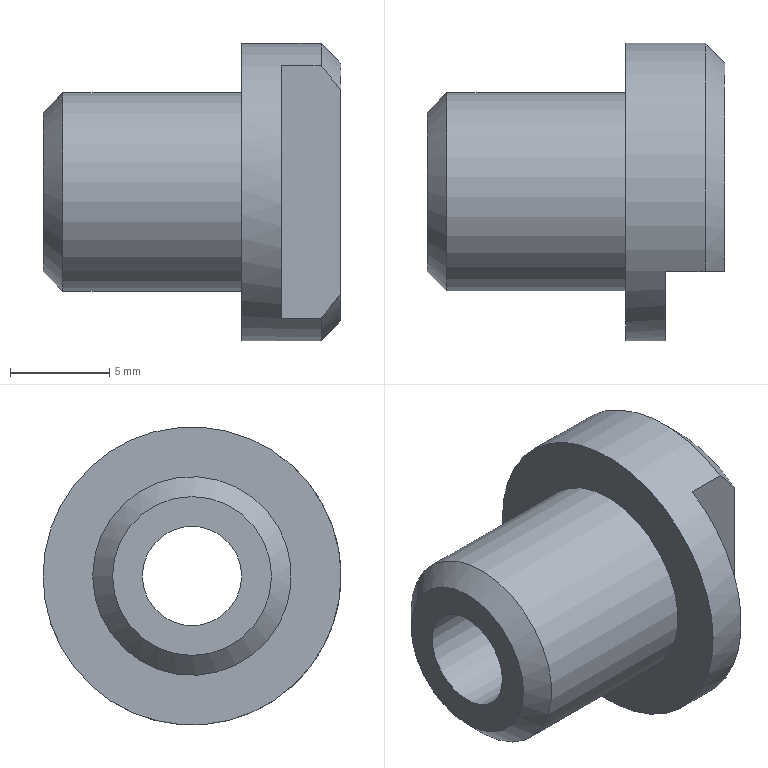Component | NX | DRILL_BUSHING | 1 solid | 10 faces | box 15 x 15 x 15 mm | volume 1250 mm3 | plane 5 | cylinder 3 | cone 2 | commonest cylinder face diameters 10 x1 15 x1 5 x1
STEP:
#1=CARTESIAN_POINT('',(0.,0.,0.));
#2=DIRECTION('',(0.,0.,1.));
#3=DIRECTION('',(1.,0.,0.));
#4=AXIS2_PLACEMENT_3D('',#1,#2,#3);
#5=CARTESIAN_POINT('',(50.511,134.396,30.));
#6=VERTEX_POINT('',#5);
#7=CARTESIAN_POINT('',(50.511,129.396,30.));
#8=DIRECTION('',(1.,0.,0.));
#9=DIRECTION('',(0.,1.,0.));
#10=AXIS2_PLACEMENT_3D('',#7,#8,#9);
#11=CIRCLE('',#10,5.);
#12=CARTESIAN_POINT('',(59.511,129.396,30.));
#13=DIRECTION('',(-1.,0.,0.));
#14=DIRECTION('',(0.,-1.,0.));
#15=AXIS2_PLACEMENT_3D('',#12,#13,#14);
#16=CYLINDRICAL_SURFACE('',#15,5.);
#17=CARTESIAN_POINT('',(9.425,9.));
#18=DIRECTION('',(-1.,0.));
#19=VECTOR('',#18,1.);
#20=LINE('',#17,#19);
#21=(GEOMETRIC_REPRESENTATION_CONTEXT(2)PARAMETRIC_REPRESENTATION_CONTEXT()REPRESENTATION_CONTEXT('',''));
#22=DEFINITIONAL_REPRESENTATION('',(#20),#21);
#23=PCURVE('',#16,#22);
#24=CARTESIAN_POINT('',(50.511,129.396,30.));
#25=DIRECTION('',(1.,0.,0.));
#26=DIRECTION('',(0.,1.,0.));
#27=AXIS2_PLACEMENT_3D('',#24,#25,#26);
#28=CONICAL_SURFACE('',#27,5.,0.7854);
#29=CARTESIAN_POINT('',(0.,0.));
#30=DIRECTION('',(1.,0.));
#31=VECTOR('',#30,1.);
#32=LINE('',#29,#31);
#33=(GEOMETRIC_REPRESENTATION_CONTEXT(2)PARAMETRIC_REPRESENTATION_CONTEXT()REPRESENTATION_CONTEXT('',''));
#34=DEFINITIONAL_REPRESENTATION('',(#32),#33);
#35=PCURVE('',#28,#34);
#36=SURFACE_CURVE('',#11,(#23,#35),.PCURVE_S1.);
#37=EDGE_CURVE('',#6,#6,#36,.T.);
#38=ORIENTED_EDGE('',*,*,#37,.T.);
#39=CARTESIAN_POINT('',(59.511,134.396,30.));
#40=VERTEX_POINT('',#39);
#41=CARTESIAN_POINT('',(59.511,134.396,30.));
#42=CARTESIAN_POINT('',(50.511,134.396,30.));
#43=B_SPLINE_CURVE_WITH_KNOTS('',1,(#41,#42),.UNSPECIFIED.,.F.,.F.,(2,2),(0.,9.),.PIECEWISE_BEZIER_KNOTS.);
#44=CARTESIAN_POINT('',(3.142,0.));
#45=DIRECTION('',(0.,1.));
#46=VECTOR('',#45,1.);
#47=LINE('',#44,#46);
#48=(GEOMETRIC_REPRESENTATION_CONTEXT(2)PARAMETRIC_REPRESENTATION_CONTEXT()REPRESENTATION_CONTEXT('',''));
#49=DEFINITIONAL_REPRESENTATION('',(#47),#48);
#50=PCURVE('',#16,#49);
#51=CARTESIAN_POINT('',(9.425,0.));
#52=DIRECTION('',(0.,1.));
#53=VECTOR('',#52,1.);
#54=LINE('',#51,#53);
#55=(GEOMETRIC_REPRESENTATION_CONTEXT(2)PARAMETRIC_REPRESENTATION_CONTEXT()REPRESENTATION_CONTEXT('',''));
#56=DEFINITIONAL_REPRESENTATION('',(#54),#55);
#57=PCURVE('',#16,#56);
#58=SEAM_CURVE('',#43,(#50,#57),.PCURVE_S1.);
#59=EDGE_CURVE('',#40,#6,#58,.T.);
#60=ORIENTED_EDGE('',*,*,#59,.F.);
#61=CARTESIAN_POINT('',(59.511,129.396,30.));
#62=DIRECTION('',(1.,0.,0.));
#63=DIRECTION('',(0.,1.,0.));
#64=AXIS2_PLACEMENT_3D('',#61,#62,#63);
#65=CIRCLE('',#64,5.);
#66=CARTESIAN_POINT('',(9.425,0.));
#67=DIRECTION('',(-1.,0.));
#68=VECTOR('',#67,1.);
#69=LINE('',#66,#68);
#70=(GEOMETRIC_REPRESENTATION_CONTEXT(2)PARAMETRIC_REPRESENTATION_CONTEXT()REPRESENTATION_CONTEXT('',''));
#71=DEFINITIONAL_REPRESENTATION('',(#69),#70);
#72=PCURVE('',#16,#71);
#73=CARTESIAN_POINT('',(59.511,129.396,30.));
#74=DIRECTION('',(1.,0.,0.));
#75=DIRECTION('',(0.,1.,0.));
#76=AXIS2_PLACEMENT_3D('',#73,#74,#75);
#77=PLANE('',#76);
#78=CARTESIAN_POINT('',(0.,0.));
#79=DIRECTION('',(1.,0.));
#80=AXIS2_PLACEMENT_2D('',#78,#79);
#81=CIRCLE('',#80,5.);
#82=(GEOMETRIC_REPRESENTATION_CONTEXT(2)PARAMETRIC_REPRESENTATION_CONTEXT()REPRESENTATION_CONTEXT('',''));
#83=DEFINITIONAL_REPRESENTATION('',(#81),#82);
#84=PCURVE('',#77,#83);
#85=SURFACE_CURVE('',#65,(#72,#84),.PCURVE_S1.);
#86=EDGE_CURVE('',#40,#40,#85,.T.);
#87=ORIENTED_EDGE('',*,*,#86,.F.);
#88=ORIENTED_EDGE('',*,*,#59,.T.);
#89=EDGE_LOOP('',(#38,#60,#87,#88));
#90=FACE_BOUND('',#89,.T.);
#91=ADVANCED_FACE('',(#90),#16,.T.);
#92=CARTESIAN_POINT('',(49.511,133.396,30.));
#93=VERTEX_POINT('',#92);
#94=CARTESIAN_POINT('',(49.511,129.396,30.));
#95=DIRECTION('',(-1.,0.,0.));
#96=DIRECTION('',(0.,1.,0.));
#97=AXIS2_PLACEMENT_3D('',#94,#95,#96);
#98=CIRCLE('',#97,4.);
#99=CARTESIAN_POINT('',(49.511,129.396,30.));
#100=DIRECTION('',(1.,0.,0.));
#101=DIRECTION('',(0.,1.,0.));
#102=AXIS2_PLACEMENT_3D('',#99,#100,#101);
#103=PLANE('',#102);
#104=CARTESIAN_POINT('',(4.,0.));
#105=CARTESIAN_POINT('',(4.,-6.928));
#106=CARTESIAN_POINT('',(-2.,-3.464));
#107=CARTESIAN_POINT('',(-8.,-0.));
#108=CARTESIAN_POINT('',(-2.,3.464));
#109=CARTESIAN_POINT('',(4.,6.928));
#110=CARTESIAN_POINT('',(4.,0.));
#111=(BOUNDED_CURVE()B_SPLINE_CURVE(2,(#104,#105,#106,#107,#108,#109,#110),.UNSPECIFIED.,.T.,.F.)B_SPLINE_CURVE_WITH_KNOTS((1,2,2,2,2,1),(-2.094,0.,2.094,4.189,6.283,8.378),.UNSPECIFIED.)CURVE()GEOMETRIC_REPRESENTATION_ITEM()RATIONAL_B_SPLINE_CURVE((1.,0.5,1.,0.5,1.,0.5,1.))REPRESENTATION_ITEM(''));
#112=(GEOMETRIC_REPRESENTATION_CONTEXT(2)PARAMETRIC_REPRESENTATION_CONTEXT()REPRESENTATION_CONTEXT('',''));
#113=DEFINITIONAL_REPRESENTATION('',(#111),#112);
#114=PCURVE('',#103,#113);
#115=CARTESIAN_POINT('',(6.283,-1.));
#116=DIRECTION('',(-1.,0.));
#117=VECTOR('',#116,1.);
#118=LINE('',#115,#117);
#119=(GEOMETRIC_REPRESENTATION_CONTEXT(2)PARAMETRIC_REPRESENTATION_CONTEXT()REPRESENTATION_CONTEXT('',''));
#120=DEFINITIONAL_REPRESENTATION('',(#118),#119);
#121=PCURVE('',#28,#120);
#122=SURFACE_CURVE('',#98,(#114,#121),.PCURVE_S1.);
#123=EDGE_CURVE('',#93,#93,#122,.T.);
#124=ORIENTED_EDGE('',*,*,#123,.T.);
#125=EDGE_LOOP('',(#124));
#126=FACE_BOUND('',#125,.T.);
#127=CARTESIAN_POINT('',(49.511,131.896,30.));
#128=VERTEX_POINT('',#127);
#129=CARTESIAN_POINT('',(49.511,129.396,30.));
#130=DIRECTION('',(1.,0.,0.));
#131=DIRECTION('',(0.,1.,0.));
#132=AXIS2_PLACEMENT_3D('',#129,#130,#131);
#133=CIRCLE('',#132,2.5);
#134=CARTESIAN_POINT('',(0.,0.));
#135=DIRECTION('',(1.,0.));
#136=AXIS2_PLACEMENT_2D('',#134,#135);
#137=CIRCLE('',#136,2.5);
#138=(GEOMETRIC_REPRESENTATION_CONTEXT(2)PARAMETRIC_REPRESENTATION_CONTEXT()REPRESENTATION_CONTEXT('',''));
#139=DEFINITIONAL_REPRESENTATION('',(#137),#138);
#140=PCURVE('',#103,#139);
#141=CARTESIAN_POINT('',(46.211,129.396,30.));
#142=DIRECTION('',(1.,0.,0.));
#143=DIRECTION('',(0.,1.,0.));
#144=AXIS2_PLACEMENT_3D('',#141,#142,#143);
#145=CYLINDRICAL_SURFACE('',#144,2.5);
#146=CARTESIAN_POINT('',(0.,3.3));
#147=DIRECTION('',(1.,0.));
#148=VECTOR('',#147,1.);
#149=LINE('',#146,#148);
#150=(GEOMETRIC_REPRESENTATION_CONTEXT(2)PARAMETRIC_REPRESENTATION_CONTEXT()REPRESENTATION_CONTEXT('',''));
#151=DEFINITIONAL_REPRESENTATION('',(#149),#150);
#152=PCURVE('',#145,#151);
#153=SURFACE_CURVE('',#133,(#140,#152),.PCURVE_S1.);
#154=EDGE_CURVE('',#128,#128,#153,.T.);
#155=ORIENTED_EDGE('',*,*,#154,.T.);
#156=EDGE_LOOP('',(#155));
#157=FACE_BOUND('',#156,.T.);
#158=ADVANCED_FACE('',(#126,#157),#103,.F.);
#159=CARTESIAN_POINT('',(63.511,125.396,36.344));
#160=VERTEX_POINT('',#159);
#161=CARTESIAN_POINT('',(63.511,125.396,23.656));
#162=VERTEX_POINT('',#161);
#163=CARTESIAN_POINT('',(63.511,129.396,30.));
#164=DIRECTION('',(-1.,0.,0.));
#165=DIRECTION('',(0.,1.,0.));
#166=AXIS2_PLACEMENT_3D('',#163,#164,#165);
#167=CIRCLE('',#166,7.5);
#168=CARTESIAN_POINT('',(64.511,129.396,30.));
#169=DIRECTION('',(-1.,0.,0.));
#170=DIRECTION('',(0.,-1.,0.));
#171=AXIS2_PLACEMENT_3D('',#168,#169,#170);
#172=CYLINDRICAL_SURFACE('',#171,7.5);
#173=CARTESIAN_POINT('',(-3.142,1.));
#174=DIRECTION('',(1.,0.));
#175=VECTOR('',#174,1.);
#176=LINE('',#173,#175);
#177=(GEOMETRIC_REPRESENTATION_CONTEXT(2)PARAMETRIC_REPRESENTATION_CONTEXT()REPRESENTATION_CONTEXT('',''));
#178=DEFINITIONAL_REPRESENTATION('',(#176),#177);
#179=PCURVE('',#172,#178);
#180=CARTESIAN_POINT('',(64.511,129.396,30.));
#181=DIRECTION('',(-1.,0.,0.));
#182=DIRECTION('',(0.,-1.,0.));
#183=AXIS2_PLACEMENT_3D('',#180,#181,#182);
#184=CONICAL_SURFACE('',#183,6.5,0.7854);
#185=CARTESIAN_POINT('',(-3.142,1.));
#186=DIRECTION('',(1.,0.));
#187=VECTOR('',#186,1.);
#188=LINE('',#185,#187);
#189=(GEOMETRIC_REPRESENTATION_CONTEXT(2)PARAMETRIC_REPRESENTATION_CONTEXT()REPRESENTATION_CONTEXT('',''));
#190=DEFINITIONAL_REPRESENTATION('',(#188),#189);
#191=PCURVE('',#184,#190);
#192=SURFACE_CURVE('',#167,(#179,#191),.PCURVE_S1.);
#193=EDGE_CURVE('',#160,#162,#192,.T.);
#194=ORIENTED_EDGE('',*,*,#193,.T.);
#195=CARTESIAN_POINT('',(61.511,125.396,23.656));
#196=VERTEX_POINT('',#195);
#197=CARTESIAN_POINT('',(64.511,125.396,23.656));
#198=DIRECTION('',(-1.,0.,0.));
#199=VECTOR('',#198,1.);
#200=LINE('',#197,#199);
#201=CARTESIAN_POINT('',(5.275,0.));
#202=DIRECTION('',(0.,1.));
#203=VECTOR('',#202,1.);
#204=LINE('',#201,#203);
#205=(GEOMETRIC_REPRESENTATION_CONTEXT(2)PARAMETRIC_REPRESENTATION_CONTEXT()REPRESENTATION_CONTEXT('',''));
#206=DEFINITIONAL_REPRESENTATION('',(#204),#205);
#207=PCURVE('',#172,#206);
#208=CARTESIAN_POINT('',(61.511,125.396,22.2));
#209=DIRECTION('',(0.,1.,0.));
#210=DIRECTION('',(0.,-0.,1.));
#211=AXIS2_PLACEMENT_3D('',#208,#209,#210);
#212=PLANE('',#211);
#213=CARTESIAN_POINT('',(1.456,3.));
#214=DIRECTION('',(0.,-1.));
#215=VECTOR('',#214,1.);
#216=LINE('',#213,#215);
#217=(GEOMETRIC_REPRESENTATION_CONTEXT(2)PARAMETRIC_REPRESENTATION_CONTEXT()REPRESENTATION_CONTEXT('',''));
#218=DEFINITIONAL_REPRESENTATION('',(#216),#217);
#219=PCURVE('',#212,#218);
#220=SURFACE_CURVE('',#200,(#207,#219),.PCURVE_S1.);
#221=EDGE_CURVE('',#162,#196,#220,.T.);
#222=ORIENTED_EDGE('',*,*,#221,.T.);
#223=CARTESIAN_POINT('',(61.511,125.396,36.344));
#224=VERTEX_POINT('',#223);
#225=CARTESIAN_POINT('',(61.511,129.396,30.));
#226=DIRECTION('',(1.,0.,0.));
#227=DIRECTION('',(0.,1.,0.));
#228=AXIS2_PLACEMENT_3D('',#225,#226,#227);
#229=CIRCLE('',#228,7.5);
#230=CARTESIAN_POINT('',(9.425,3.));
#231=DIRECTION('',(-1.,0.));
#232=VECTOR('',#231,1.);
#233=LINE('',#230,#232);
#234=(GEOMETRIC_REPRESENTATION_CONTEXT(2)PARAMETRIC_REPRESENTATION_CONTEXT()REPRESENTATION_CONTEXT('',''));
#235=DEFINITIONAL_REPRESENTATION('',(#233),#234);
#236=PCURVE('',#172,#235);
#237=CARTESIAN_POINT('',(61.511,129.396,30.));
#238=DIRECTION('',(1.,0.,0.));
#239=DIRECTION('',(0.,1.,0.));
#240=AXIS2_PLACEMENT_3D('',#237,#238,#239);
#241=PLANE('',#240);
#242=CARTESIAN_POINT('',(0.,0.));
#243=DIRECTION('',(1.,0.));
#244=AXIS2_PLACEMENT_2D('',#242,#243);
#245=CIRCLE('',#244,7.5);
#246=(GEOMETRIC_REPRESENTATION_CONTEXT(2)PARAMETRIC_REPRESENTATION_CONTEXT()REPRESENTATION_CONTEXT('',''));
#247=DEFINITIONAL_REPRESENTATION('',(#245),#246);
#248=PCURVE('',#241,#247);
#249=SURFACE_CURVE('',#229,(#236,#248),.PCURVE_S1.);
#250=EDGE_CURVE('',#224,#196,#249,.T.);
#251=ORIENTED_EDGE('',*,*,#250,.F.);
#252=CARTESIAN_POINT('',(59.511,125.396,36.344));
#253=VERTEX_POINT('',#252);
#254=CARTESIAN_POINT('',(61.511,125.396,36.344));
#255=CARTESIAN_POINT('',(59.511,125.396,36.344));
#256=B_SPLINE_CURVE_WITH_KNOTS('',1,(#254,#255),.UNSPECIFIED.,.F.,.F.,(2,2),(3.,5.),.PIECEWISE_BEZIER_KNOTS.);
#257=CARTESIAN_POINT('',(7.291,0.));
#258=DIRECTION('',(0.,1.));
#259=VECTOR('',#258,1.);
#260=LINE('',#257,#259);
#261=(GEOMETRIC_REPRESENTATION_CONTEXT(2)PARAMETRIC_REPRESENTATION_CONTEXT()REPRESENTATION_CONTEXT('',''));
#262=DEFINITIONAL_REPRESENTATION('',(#260),#261);
#263=PCURVE('',#172,#262);
#264=CARTESIAN_POINT('',(1.008,0.));
#265=DIRECTION('',(0.,1.));
#266=VECTOR('',#265,1.);
#267=LINE('',#264,#266);
#268=(GEOMETRIC_REPRESENTATION_CONTEXT(2)PARAMETRIC_REPRESENTATION_CONTEXT()REPRESENTATION_CONTEXT('',''));
#269=DEFINITIONAL_REPRESENTATION('',(#267),#268);
#270=PCURVE('',#172,#269);
#271=SEAM_CURVE('',#256,(#263,#270),.PCURVE_S1.);
#272=EDGE_CURVE('',#224,#253,#271,.T.);
#273=ORIENTED_EDGE('',*,*,#272,.T.);
#274=CARTESIAN_POINT('',(59.511,136.896,30.));
#275=VERTEX_POINT('',#274);
#276=CARTESIAN_POINT('',(59.511,129.396,30.));
#277=DIRECTION('',(1.,0.,0.));
#278=DIRECTION('',(0.,1.,0.));
#279=AXIS2_PLACEMENT_3D('',#276,#277,#278);
#280=CIRCLE('',#279,7.5);
#281=CARTESIAN_POINT('',(9.425,5.));
#282=DIRECTION('',(-1.,0.));
#283=VECTOR('',#282,1.);
#284=LINE('',#281,#283);
#285=(GEOMETRIC_REPRESENTATION_CONTEXT(2)PARAMETRIC_REPRESENTATION_CONTEXT()REPRESENTATION_CONTEXT('',''));
#286=DEFINITIONAL_REPRESENTATION('',(#284),#285);
#287=PCURVE('',#172,#286);
#288=CARTESIAN_POINT('',(0.,0.));
#289=DIRECTION('',(1.,0.));
#290=AXIS2_PLACEMENT_2D('',#288,#289);
#291=CIRCLE('',#290,7.5);
#292=(GEOMETRIC_REPRESENTATION_CONTEXT(2)PARAMETRIC_REPRESENTATION_CONTEXT()REPRESENTATION_CONTEXT('',''));
#293=DEFINITIONAL_REPRESENTATION('',(#291),#292);
#294=PCURVE('',#77,#293);
#295=SURFACE_CURVE('',#280,(#287,#294),.PCURVE_S1.);
#296=EDGE_CURVE('',#253,#275,#295,.T.);
#297=ORIENTED_EDGE('',*,*,#296,.T.);
#298=CARTESIAN_POINT('',(59.511,129.396,30.));
#299=DIRECTION('',(1.,0.,0.));
#300=DIRECTION('',(0.,1.,0.));
#301=AXIS2_PLACEMENT_3D('',#298,#299,#300);
#302=CIRCLE('',#301,7.5);
#303=CARTESIAN_POINT('',(3.142,5.));
#304=DIRECTION('',(-1.,0.));
#305=VECTOR('',#304,1.);
#306=LINE('',#303,#305);
#307=(GEOMETRIC_REPRESENTATION_CONTEXT(2)PARAMETRIC_REPRESENTATION_CONTEXT()REPRESENTATION_CONTEXT('',''));
#308=DEFINITIONAL_REPRESENTATION('',(#306),#307);
#309=PCURVE('',#172,#308);
#310=CARTESIAN_POINT('',(0.,0.));
#311=DIRECTION('',(1.,0.));
#312=AXIS2_PLACEMENT_2D('',#310,#311);
#313=CIRCLE('',#312,7.5);
#314=(GEOMETRIC_REPRESENTATION_CONTEXT(2)PARAMETRIC_REPRESENTATION_CONTEXT()REPRESENTATION_CONTEXT('',''));
#315=DEFINITIONAL_REPRESENTATION('',(#313),#314);
#316=PCURVE('',#77,#315);
#317=SURFACE_CURVE('',#302,(#309,#316),.PCURVE_S1.);
#318=EDGE_CURVE('',#275,#253,#317,.T.);
#319=ORIENTED_EDGE('',*,*,#318,.T.);
#320=ORIENTED_EDGE('',*,*,#272,.F.);
#321=CARTESIAN_POINT('',(64.511,125.396,36.344));
#322=DIRECTION('',(1.,0.,0.));
#323=VECTOR('',#322,1.);
#324=LINE('',#321,#323);
#325=CARTESIAN_POINT('',(1.008,0.));
#326=DIRECTION('',(0.,-1.));
#327=VECTOR('',#326,1.);
#328=LINE('',#325,#327);
#329=(GEOMETRIC_REPRESENTATION_CONTEXT(2)PARAMETRIC_REPRESENTATION_CONTEXT()REPRESENTATION_CONTEXT('',''));
#330=DEFINITIONAL_REPRESENTATION('',(#328),#329);
#331=PCURVE('',#172,#330);
#332=CARTESIAN_POINT('',(14.144,3.));
#333=DIRECTION('',(0.,1.));
#334=VECTOR('',#333,1.);
#335=LINE('',#332,#334);
#336=(GEOMETRIC_REPRESENTATION_CONTEXT(2)PARAMETRIC_REPRESENTATION_CONTEXT()REPRESENTATION_CONTEXT('',''));
#337=DEFINITIONAL_REPRESENTATION('',(#335),#336);
#338=PCURVE('',#212,#337);
#339=SURFACE_CURVE('',#324,(#331,#338),.PCURVE_S1.);
#340=EDGE_CURVE('',#224,#160,#339,.T.);
#341=ORIENTED_EDGE('',*,*,#340,.T.);
#342=EDGE_LOOP('',(#194,#222,#251,#273,#297,#319,#320,#341));
#343=FACE_BOUND('',#342,.T.);
#344=ADVANCED_FACE('',(#343),#172,.T.);
#345=CARTESIAN_POINT('',(64.511,125.396,24.877));
#346=VERTEX_POINT('',#345);
#347=CARTESIAN_POINT('',(64.511,125.396,35.123));
#348=VERTEX_POINT('',#347);
#349=CARTESIAN_POINT('',(64.511,125.396,22.2));
#350=DIRECTION('',(0.,-0.,1.));
#351=VECTOR('',#350,1.);
#352=LINE('',#349,#351);
#353=CARTESIAN_POINT('',(64.511,129.396,30.));
#354=DIRECTION('',(1.,0.,0.));
#355=DIRECTION('',(0.,1.,0.));
#356=AXIS2_PLACEMENT_3D('',#353,#354,#355);
#357=PLANE('',#356);
#358=CARTESIAN_POINT('',(-4.,-7.8));
#359=DIRECTION('',(-0.,1.));
#360=VECTOR('',#359,1.);
#361=LINE('',#358,#360);
#362=(GEOMETRIC_REPRESENTATION_CONTEXT(2)PARAMETRIC_REPRESENTATION_CONTEXT()REPRESENTATION_CONTEXT('',''));
#363=DEFINITIONAL_REPRESENTATION('',(#361),#362);
#364=PCURVE('',#357,#363);
#365=CARTESIAN_POINT('',(0.,3.));
#366=DIRECTION('',(1.,0.));
#367=VECTOR('',#366,1.);
#368=LINE('',#365,#367);
#369=(GEOMETRIC_REPRESENTATION_CONTEXT(2)PARAMETRIC_REPRESENTATION_CONTEXT()REPRESENTATION_CONTEXT('',''));
#370=DEFINITIONAL_REPRESENTATION('',(#368),#369);
#371=PCURVE('',#212,#370);
#372=SURFACE_CURVE('',#352,(#364,#371),.PCURVE_S1.);
#373=EDGE_CURVE('',#346,#348,#372,.T.);
#374=ORIENTED_EDGE('',*,*,#373,.F.);
#375=CARTESIAN_POINT('',(64.511,129.396,30.));
#376=DIRECTION('',(1.,0.,0.));
#377=DIRECTION('',(0.,1.,0.));
#378=AXIS2_PLACEMENT_3D('',#375,#376,#377);
#379=CIRCLE('',#378,6.5);
#380=CARTESIAN_POINT('',(0.,0.));
#381=DIRECTION('',(1.,0.));
#382=AXIS2_PLACEMENT_2D('',#380,#381);
#383=CIRCLE('',#382,6.5);
#384=(GEOMETRIC_REPRESENTATION_CONTEXT(2)PARAMETRIC_REPRESENTATION_CONTEXT()REPRESENTATION_CONTEXT('',''));
#385=DEFINITIONAL_REPRESENTATION('',(#383),#384);
#386=PCURVE('',#357,#385);
#387=CARTESIAN_POINT('',(9.425,0.));
#388=DIRECTION('',(-1.,-0.));
#389=VECTOR('',#388,1.);
#390=LINE('',#387,#389);
#391=(GEOMETRIC_REPRESENTATION_CONTEXT(2)PARAMETRIC_REPRESENTATION_CONTEXT()REPRESENTATION_CONTEXT('',''));
#392=DEFINITIONAL_REPRESENTATION('',(#390),#391);
#393=PCURVE('',#184,#392);
#394=SURFACE_CURVE('',#379,(#386,#393),.PCURVE_S1.);
#395=EDGE_CURVE('',#346,#348,#394,.T.);
#396=ORIENTED_EDGE('',*,*,#395,.T.);
#397=EDGE_LOOP('',(#374,#396));
#398=FACE_BOUND('',#397,.T.);
#399=CARTESIAN_POINT('',(64.511,131.896,30.));
#400=VERTEX_POINT('',#399);
#401=CARTESIAN_POINT('',(64.511,129.396,30.));
#402=DIRECTION('',(1.,0.,0.));
#403=DIRECTION('',(0.,1.,0.));
#404=AXIS2_PLACEMENT_3D('',#401,#402,#403);
#405=CIRCLE('',#404,2.5);
#406=CARTESIAN_POINT('',(0.,0.));
#407=DIRECTION('',(1.,0.));
#408=AXIS2_PLACEMENT_2D('',#406,#407);
#409=CIRCLE('',#408,2.5);
#410=(GEOMETRIC_REPRESENTATION_CONTEXT(2)PARAMETRIC_REPRESENTATION_CONTEXT()REPRESENTATION_CONTEXT('',''));
#411=DEFINITIONAL_REPRESENTATION('',(#409),#410);
#412=PCURVE('',#357,#411);
#413=CARTESIAN_POINT('',(0.,18.3));
#414=DIRECTION('',(1.,0.));
#415=VECTOR('',#414,1.);
#416=LINE('',#413,#415);
#417=(GEOMETRIC_REPRESENTATION_CONTEXT(2)PARAMETRIC_REPRESENTATION_CONTEXT()REPRESENTATION_CONTEXT('',''));
#418=DEFINITIONAL_REPRESENTATION('',(#416),#417);
#419=PCURVE('',#145,#418);
#420=SURFACE_CURVE('',#405,(#412,#419),.PCURVE_S1.);
#421=EDGE_CURVE('',#400,#400,#420,.T.);
#422=ORIENTED_EDGE('',*,*,#421,.F.);
#423=EDGE_LOOP('',(#422));
#424=FACE_BOUND('',#423,.T.);
#425=ADVANCED_FACE('',(#398,#424),#357,.T.);
#426=ORIENTED_EDGE('',*,*,#86,.T.);
#427=EDGE_LOOP('',(#426));
#428=FACE_BOUND('',#427,.T.);
#429=ORIENTED_EDGE('',*,*,#318,.F.);
#430=ORIENTED_EDGE('',*,*,#296,.F.);
#431=EDGE_LOOP('',(#429,#430));
#432=FACE_BOUND('',#431,.T.);
#433=ADVANCED_FACE('',(#428,#432),#77,.F.);
#434=ORIENTED_EDGE('',*,*,#421,.F.);
#435=CARTESIAN_POINT('',(49.511,131.896,30.));
#436=CARTESIAN_POINT('',(64.511,131.896,30.));
#437=B_SPLINE_CURVE_WITH_KNOTS('',1,(#435,#436),.UNSPECIFIED.,.F.,.F.,(2,2),(3.3,18.3),.PIECEWISE_BEZIER_KNOTS.);
#438=CARTESIAN_POINT('',(0.,0.));
#439=DIRECTION('',(0.,1.));
#440=VECTOR('',#439,1.);
#441=LINE('',#438,#440);
#442=(GEOMETRIC_REPRESENTATION_CONTEXT(2)PARAMETRIC_REPRESENTATION_CONTEXT()REPRESENTATION_CONTEXT('',''));
#443=DEFINITIONAL_REPRESENTATION('',(#441),#442);
#444=PCURVE('',#145,#443);
#445=CARTESIAN_POINT('',(6.283,0.));
#446=DIRECTION('',(0.,1.));
#447=VECTOR('',#446,1.);
#448=LINE('',#445,#447);
#449=(GEOMETRIC_REPRESENTATION_CONTEXT(2)PARAMETRIC_REPRESENTATION_CONTEXT()REPRESENTATION_CONTEXT('',''));
#450=DEFINITIONAL_REPRESENTATION('',(#448),#449);
#451=PCURVE('',#145,#450);
#452=SEAM_CURVE('',#437,(#444,#451),.PCURVE_S1.);
#453=EDGE_CURVE('',#128,#400,#452,.T.);
#454=ORIENTED_EDGE('',*,*,#453,.F.);
#455=ORIENTED_EDGE('',*,*,#154,.T.);
#456=ORIENTED_EDGE('',*,*,#453,.T.);
#457=EDGE_LOOP('',(#434,#454,#455,#456));
#458=FACE_BOUND('',#457,.F.);
#459=ADVANCED_FACE('',(#458),#145,.F.);
#460=ORIENTED_EDGE('',*,*,#123,.F.);
#461=CARTESIAN_POINT('',(49.511,133.396,30.));
#462=CARTESIAN_POINT('',(50.511,134.396,30.));
#463=B_SPLINE_CURVE_WITH_KNOTS('',1,(#461,#462),.UNSPECIFIED.,.F.,.F.,(2,2),(-1.414,0.),.PIECEWISE_BEZIER_KNOTS.);
#464=CARTESIAN_POINT('',(6.283,0.));
#465=DIRECTION('',(0.,1.));
#466=VECTOR('',#465,1.);
#467=LINE('',#464,#466);
#468=(GEOMETRIC_REPRESENTATION_CONTEXT(2)PARAMETRIC_REPRESENTATION_CONTEXT()REPRESENTATION_CONTEXT('',''));
#469=DEFINITIONAL_REPRESENTATION('',(#467),#468);
#470=PCURVE('',#28,#469);
#471=CARTESIAN_POINT('',(0.,0.));
#472=DIRECTION('',(0.,1.));
#473=VECTOR('',#472,1.);
#474=LINE('',#471,#473);
#475=(GEOMETRIC_REPRESENTATION_CONTEXT(2)PARAMETRIC_REPRESENTATION_CONTEXT()REPRESENTATION_CONTEXT('',''));
#476=DEFINITIONAL_REPRESENTATION('',(#474),#475);
#477=PCURVE('',#28,#476);
#478=SEAM_CURVE('',#463,(#470,#477),.PCURVE_S1.);
#479=EDGE_CURVE('',#93,#6,#478,.T.);
#480=ORIENTED_EDGE('',*,*,#479,.T.);
#481=ORIENTED_EDGE('',*,*,#37,.F.);
#482=ORIENTED_EDGE('',*,*,#479,.F.);
#483=EDGE_LOOP('',(#460,#480,#481,#482));
#484=FACE_BOUND('',#483,.T.);
#485=ADVANCED_FACE('',(#484),#28,.T.);
#486=CARTESIAN_POINT('',(63.511,125.396,23.656));
#487=CARTESIAN_POINT('',(63.851,125.396,24.058));
#488=CARTESIAN_POINT('',(64.185,125.396,24.464));
#489=CARTESIAN_POINT('',(64.511,125.396,24.877));
#490=B_SPLINE_CURVE_WITH_KNOTS('',3,(#486,#487,#488,#489),.UNSPECIFIED.,.F.,.F.,(4,4),(0.,1.),.PIECEWISE_BEZIER_KNOTS.);
#491=CARTESIAN_POINT('',(5.275,1.));
#492=CARTESIAN_POINT('',(5.375,0.));
#493=B_SPLINE_CURVE_WITH_KNOTS('',1,(#491,#492),.UNSPECIFIED.,.F.,.F.,(2,2),(0.,1.),.PIECEWISE_BEZIER_KNOTS.);
#494=(GEOMETRIC_REPRESENTATION_CONTEXT(2)PARAMETRIC_REPRESENTATION_CONTEXT()REPRESENTATION_CONTEXT('',''));
#495=DEFINITIONAL_REPRESENTATION('',(#493),#494);
#496=PCURVE('',#184,#495);
#497=CARTESIAN_POINT('',(1.456,2.));
#498=CARTESIAN_POINT('',(1.858,2.34));
#499=CARTESIAN_POINT('',(2.264,2.675));
#500=CARTESIAN_POINT('',(2.677,3.));
#501=B_SPLINE_CURVE_WITH_KNOTS('',3,(#497,#498,#499,#500),.UNSPECIFIED.,.F.,.F.,(4,4),(0.,1.),.PIECEWISE_BEZIER_KNOTS.);
#502=(GEOMETRIC_REPRESENTATION_CONTEXT(2)PARAMETRIC_REPRESENTATION_CONTEXT()REPRESENTATION_CONTEXT('',''));
#503=DEFINITIONAL_REPRESENTATION('',(#501),#502);
#504=PCURVE('',#212,#503);
#505=SURFACE_CURVE('',#490,(#496,#504),.PCURVE_S1.);
#506=EDGE_CURVE('',#162,#346,#505,.T.);
#507=ORIENTED_EDGE('',*,*,#506,.F.);
#508=ORIENTED_EDGE('',*,*,#193,.F.);
#509=CARTESIAN_POINT('',(64.511,125.396,35.123));
#510=CARTESIAN_POINT('',(64.185,125.396,35.537));
#511=CARTESIAN_POINT('',(63.85,125.396,35.943));
#512=CARTESIAN_POINT('',(63.511,125.396,36.344));
#513=B_SPLINE_CURVE_WITH_KNOTS('',3,(#509,#510,#511,#512),.UNSPECIFIED.,.F.,.F.,(4,4),(0.,1.),.PIECEWISE_BEZIER_KNOTS.);
#514=CARTESIAN_POINT('',(0.9079,-0.));
#515=CARTESIAN_POINT('',(1.008,1.));
#516=B_SPLINE_CURVE_WITH_KNOTS('',1,(#514,#515),.UNSPECIFIED.,.F.,.F.,(2,2),(0.,1.),.PIECEWISE_BEZIER_KNOTS.);
#517=(GEOMETRIC_REPRESENTATION_CONTEXT(2)PARAMETRIC_REPRESENTATION_CONTEXT()REPRESENTATION_CONTEXT('',''));
#518=DEFINITIONAL_REPRESENTATION('',(#516),#517);
#519=PCURVE('',#184,#518);
#520=CARTESIAN_POINT('',(12.923,3.));
#521=CARTESIAN_POINT('',(13.337,2.674));
#522=CARTESIAN_POINT('',(13.743,2.339));
#523=CARTESIAN_POINT('',(14.144,2.));
#524=B_SPLINE_CURVE_WITH_KNOTS('',3,(#520,#521,#522,#523),.UNSPECIFIED.,.F.,.F.,(4,4),(0.,1.),.PIECEWISE_BEZIER_KNOTS.);
#525=(GEOMETRIC_REPRESENTATION_CONTEXT(2)PARAMETRIC_REPRESENTATION_CONTEXT()REPRESENTATION_CONTEXT('',''));
#526=DEFINITIONAL_REPRESENTATION('',(#524),#525);
#527=PCURVE('',#212,#526);
#528=SURFACE_CURVE('',#513,(#519,#527),.PCURVE_S1.);
#529=EDGE_CURVE('',#348,#160,#528,.T.);
#530=ORIENTED_EDGE('',*,*,#529,.F.);
#531=ORIENTED_EDGE('',*,*,#395,.F.);
#532=EDGE_LOOP('',(#507,#508,#530,#531));
#533=FACE_BOUND('',#532,.T.);
#534=ADVANCED_FACE('',(#533),#184,.T.);
#535=ORIENTED_EDGE('',*,*,#250,.T.);
#536=CARTESIAN_POINT('',(61.511,125.396,22.2));
#537=DIRECTION('',(0.,0.,-1.));
#538=VECTOR('',#537,1.);
#539=LINE('',#536,#538);
#540=CARTESIAN_POINT('',(-4.,-7.8));
#541=DIRECTION('',(0.,-1.));
#542=VECTOR('',#541,1.);
#543=LINE('',#540,#542);
#544=(GEOMETRIC_REPRESENTATION_CONTEXT(2)PARAMETRIC_REPRESENTATION_CONTEXT()REPRESENTATION_CONTEXT('',''));
#545=DEFINITIONAL_REPRESENTATION('',(#543),#544);
#546=PCURVE('',#241,#545);
#547=CARTESIAN_POINT('',(0.,0.));
#548=DIRECTION('',(-1.,0.));
#549=VECTOR('',#548,1.);
#550=LINE('',#547,#549);
#551=(GEOMETRIC_REPRESENTATION_CONTEXT(2)PARAMETRIC_REPRESENTATION_CONTEXT()REPRESENTATION_CONTEXT('',''));
#552=DEFINITIONAL_REPRESENTATION('',(#550),#551);
#553=PCURVE('',#212,#552);
#554=SURFACE_CURVE('',#539,(#546,#553),.PCURVE_S1.);
#555=EDGE_CURVE('',#224,#196,#554,.T.);
#556=ORIENTED_EDGE('',*,*,#555,.F.);
#557=EDGE_LOOP('',(#535,#556));
#558=FACE_BOUND('',#557,.T.);
#559=ADVANCED_FACE('',(#558),#241,.T.);
#560=ORIENTED_EDGE('',*,*,#506,.T.);
#561=ORIENTED_EDGE('',*,*,#373,.T.);
#562=ORIENTED_EDGE('',*,*,#529,.T.);
#563=ORIENTED_EDGE('',*,*,#340,.F.);
#564=ORIENTED_EDGE('',*,*,#555,.T.);
#565=ORIENTED_EDGE('',*,*,#221,.F.);
#566=EDGE_LOOP('',(#560,#561,#562,#563,#564,#565));
#567=FACE_BOUND('',#566,.T.);
#568=ADVANCED_FACE('',(#567),#212,.F.);
#569=CLOSED_SHELL('',(#91,#158,#344,#425,#433,#459,#485,#534,#559,#568));
#570=MANIFOLD_SOLID_BREP('',#569);
#571=(LENGTH_UNIT()NAMED_UNIT(*)SI_UNIT(.MILLI.,.METRE.));
#572=UNCERTAINTY_MEASURE_WITH_UNIT(LENGTH_MEASURE(0.005),#571,'','');
#573=(NAMED_UNIT(*)PLANE_ANGLE_UNIT()SI_UNIT($,.RADIAN.));
#574=(NAMED_UNIT(*)SI_UNIT($,.STERADIAN.)SOLID_ANGLE_UNIT());
#575=(GEOMETRIC_REPRESENTATION_CONTEXT(3)GLOBAL_UNCERTAINTY_ASSIGNED_CONTEXT((#572))GLOBAL_UNIT_ASSIGNED_CONTEXT((#571,#573,#574))REPRESENTATION_CONTEXT('',''));
#576=ADVANCED_BREP_SHAPE_REPRESENTATION('',(#4,#570),#575);